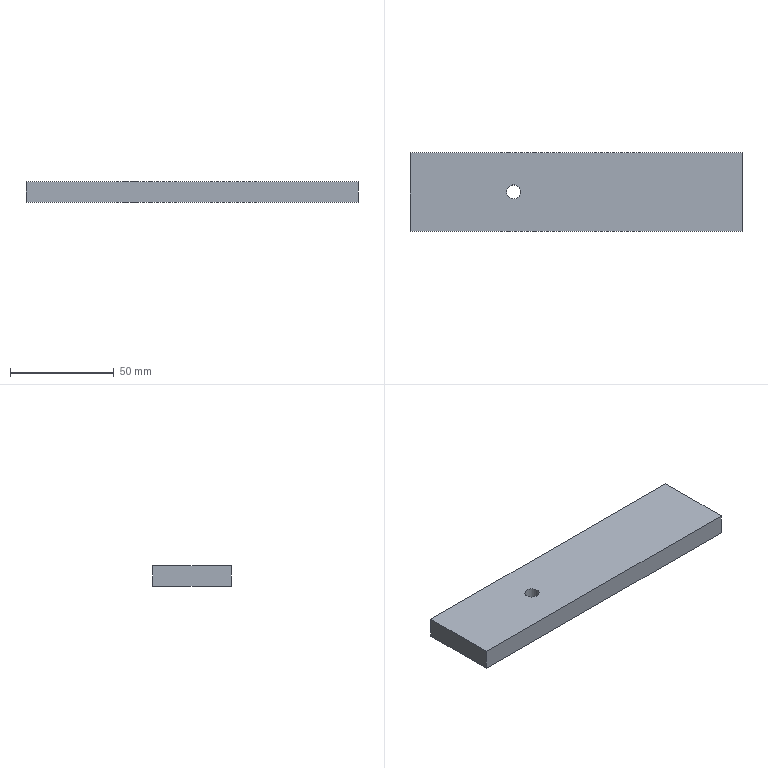Component | NX | FIXED_PLATE_11 | 1 solid | 7 faces | box 160 x 38 x 10 mm | volume 60437 mm3 | plane 6 | cylinder 1 | commonest cylinder face diameters 6.8 x1
STEP:
#1=CARTESIAN_POINT('',(0.,0.,0.));
#2=DIRECTION('',(0.,0.,1.));
#3=DIRECTION('',(1.,0.,0.));
#4=AXIS2_PLACEMENT_3D('',#1,#2,#3);
#5=CARTESIAN_POINT('',(1356.736,1345.,801.574));
#6=VERTEX_POINT('',#5);
#7=CARTESIAN_POINT('',(1356.736,1307.,801.574));
#8=VERTEX_POINT('',#7);
#9=CARTESIAN_POINT('',(1356.736,1345.,801.574));
#10=DIRECTION('',(0.,-1.,0.));
#11=VECTOR('',#10,1.);
#12=LINE('',#9,#11);
#13=CARTESIAN_POINT('',(1356.736,1345.,791.574));
#14=DIRECTION('',(-1.,0.,0.));
#15=DIRECTION('',(0.,0.,1.));
#16=AXIS2_PLACEMENT_3D('',#13,#14,#15);
#17=PLANE('',#16);
#18=CARTESIAN_POINT('',(10.,0.));
#19=DIRECTION('',(0.,-1.));
#20=VECTOR('',#19,1.);
#21=LINE('',#18,#20);
#22=(GEOMETRIC_REPRESENTATION_CONTEXT(2)PARAMETRIC_REPRESENTATION_CONTEXT()REPRESENTATION_CONTEXT('',''));
#23=DEFINITIONAL_REPRESENTATION('',(#21),#22);
#24=PCURVE('',#17,#23);
#25=CARTESIAN_POINT('',(1406.736,1326.,801.574));
#26=DIRECTION('',(0.,0.,1.));
#27=DIRECTION('',(1.,0.,0.));
#28=AXIS2_PLACEMENT_3D('',#25,#26,#27);
#29=PLANE('',#28);
#30=CARTESIAN_POINT('',(-50.,19.));
#31=DIRECTION('',(0.,-1.));
#32=VECTOR('',#31,1.);
#33=LINE('',#30,#32);
#34=(GEOMETRIC_REPRESENTATION_CONTEXT(2)PARAMETRIC_REPRESENTATION_CONTEXT()REPRESENTATION_CONTEXT('',''));
#35=DEFINITIONAL_REPRESENTATION('',(#33),#34);
#36=PCURVE('',#29,#35);
#37=SURFACE_CURVE('',#12,(#24,#36),.PCURVE_S1.);
#38=EDGE_CURVE('',#6,#8,#37,.T.);
#39=ORIENTED_EDGE('',*,*,#38,.F.);
#40=CARTESIAN_POINT('',(1356.736,1345.,791.574));
#41=VERTEX_POINT('',#40);
#42=CARTESIAN_POINT('',(1356.736,1345.,791.574));
#43=DIRECTION('',(0.,0.,1.));
#44=VECTOR('',#43,1.);
#45=LINE('',#42,#44);
#46=CARTESIAN_POINT('',(0.,0.));
#47=DIRECTION('',(1.,0.));
#48=VECTOR('',#47,1.);
#49=LINE('',#46,#48);
#50=(GEOMETRIC_REPRESENTATION_CONTEXT(2)PARAMETRIC_REPRESENTATION_CONTEXT()REPRESENTATION_CONTEXT('',''));
#51=DEFINITIONAL_REPRESENTATION('',(#49),#50);
#52=PCURVE('',#17,#51);
#53=CARTESIAN_POINT('',(1516.736,1345.,791.574));
#54=DIRECTION('',(0.,1.,0.));
#55=DIRECTION('',(0.,0.,1.));
#56=AXIS2_PLACEMENT_3D('',#53,#54,#55);
#57=PLANE('',#56);
#58=CARTESIAN_POINT('',(0.,-160.));
#59=DIRECTION('',(1.,0.));
#60=VECTOR('',#59,1.);
#61=LINE('',#58,#60);
#62=(GEOMETRIC_REPRESENTATION_CONTEXT(2)PARAMETRIC_REPRESENTATION_CONTEXT()REPRESENTATION_CONTEXT('',''));
#63=DEFINITIONAL_REPRESENTATION('',(#61),#62);
#64=PCURVE('',#57,#63);
#65=SURFACE_CURVE('',#45,(#52,#64),.PCURVE_S1.);
#66=EDGE_CURVE('',#41,#6,#65,.T.);
#67=ORIENTED_EDGE('',*,*,#66,.F.);
#68=CARTESIAN_POINT('',(1356.736,1307.,791.574));
#69=VERTEX_POINT('',#68);
#70=CARTESIAN_POINT('',(1356.736,1345.,791.574));
#71=DIRECTION('',(0.,-1.,0.));
#72=VECTOR('',#71,1.);
#73=LINE('',#70,#72);
#74=CARTESIAN_POINT('',(0.,0.));
#75=DIRECTION('',(0.,-1.));
#76=VECTOR('',#75,1.);
#77=LINE('',#74,#76);
#78=(GEOMETRIC_REPRESENTATION_CONTEXT(2)PARAMETRIC_REPRESENTATION_CONTEXT()REPRESENTATION_CONTEXT('',''));
#79=DEFINITIONAL_REPRESENTATION('',(#77),#78);
#80=PCURVE('',#17,#79);
#81=CARTESIAN_POINT('',(1406.736,1326.,791.574));
#82=DIRECTION('',(0.,0.,1.));
#83=DIRECTION('',(1.,0.,0.));
#84=AXIS2_PLACEMENT_3D('',#81,#82,#83);
#85=PLANE('',#84);
#86=CARTESIAN_POINT('',(-50.,19.));
#87=DIRECTION('',(0.,-1.));
#88=VECTOR('',#87,1.);
#89=LINE('',#86,#88);
#90=(GEOMETRIC_REPRESENTATION_CONTEXT(2)PARAMETRIC_REPRESENTATION_CONTEXT()REPRESENTATION_CONTEXT('',''));
#91=DEFINITIONAL_REPRESENTATION('',(#89),#90);
#92=PCURVE('',#85,#91);
#93=SURFACE_CURVE('',#73,(#80,#92),.PCURVE_S1.);
#94=EDGE_CURVE('',#41,#69,#93,.T.);
#95=ORIENTED_EDGE('',*,*,#94,.T.);
#96=CARTESIAN_POINT('',(1356.736,1307.,791.574));
#97=DIRECTION('',(0.,0.,1.));
#98=VECTOR('',#97,1.);
#99=LINE('',#96,#98);
#100=CARTESIAN_POINT('',(0.,-38.));
#101=DIRECTION('',(1.,0.));
#102=VECTOR('',#101,1.);
#103=LINE('',#100,#102);
#104=(GEOMETRIC_REPRESENTATION_CONTEXT(2)PARAMETRIC_REPRESENTATION_CONTEXT()REPRESENTATION_CONTEXT('',''));
#105=DEFINITIONAL_REPRESENTATION('',(#103),#104);
#106=PCURVE('',#17,#105);
#107=CARTESIAN_POINT('',(1356.736,1307.,791.574));
#108=DIRECTION('',(-0.,-1.,0.));
#109=DIRECTION('',(1.,-0.,0.));
#110=AXIS2_PLACEMENT_3D('',#107,#108,#109);
#111=PLANE('',#110);
#112=CARTESIAN_POINT('',(0.,0.));
#113=DIRECTION('',(0.,1.));
#114=VECTOR('',#113,1.);
#115=LINE('',#112,#114);
#116=(GEOMETRIC_REPRESENTATION_CONTEXT(2)PARAMETRIC_REPRESENTATION_CONTEXT()REPRESENTATION_CONTEXT('',''));
#117=DEFINITIONAL_REPRESENTATION('',(#115),#116);
#118=PCURVE('',#111,#117);
#119=SURFACE_CURVE('',#99,(#106,#118),.PCURVE_S1.);
#120=EDGE_CURVE('',#69,#8,#119,.T.);
#121=ORIENTED_EDGE('',*,*,#120,.T.);
#122=EDGE_LOOP('',(#39,#67,#95,#121));
#123=FACE_BOUND('',#122,.T.);
#124=ADVANCED_FACE('',(#123),#17,.T.);
#125=CARTESIAN_POINT('',(1516.736,1307.,801.574));
#126=VERTEX_POINT('',#125);
#127=CARTESIAN_POINT('',(1356.736,1307.,801.574));
#128=DIRECTION('',(1.,-0.,0.));
#129=VECTOR('',#128,1.);
#130=LINE('',#127,#129);
#131=CARTESIAN_POINT('',(0.,10.));
#132=DIRECTION('',(1.,0.));
#133=VECTOR('',#132,1.);
#134=LINE('',#131,#133);
#135=(GEOMETRIC_REPRESENTATION_CONTEXT(2)PARAMETRIC_REPRESENTATION_CONTEXT()REPRESENTATION_CONTEXT('',''));
#136=DEFINITIONAL_REPRESENTATION('',(#134),#135);
#137=PCURVE('',#111,#136);
#138=CARTESIAN_POINT('',(-50.,-19.));
#139=DIRECTION('',(1.,-0.));
#140=VECTOR('',#139,1.);
#141=LINE('',#138,#140);
#142=(GEOMETRIC_REPRESENTATION_CONTEXT(2)PARAMETRIC_REPRESENTATION_CONTEXT()REPRESENTATION_CONTEXT('',''));
#143=DEFINITIONAL_REPRESENTATION('',(#141),#142);
#144=PCURVE('',#29,#143);
#145=SURFACE_CURVE('',#130,(#137,#144),.PCURVE_S1.);
#146=EDGE_CURVE('',#8,#126,#145,.T.);
#147=ORIENTED_EDGE('',*,*,#146,.F.);
#148=ORIENTED_EDGE('',*,*,#120,.F.);
#149=CARTESIAN_POINT('',(1516.736,1307.,791.574));
#150=VERTEX_POINT('',#149);
#151=CARTESIAN_POINT('',(1356.736,1307.,791.574));
#152=DIRECTION('',(1.,-0.,0.));
#153=VECTOR('',#152,1.);
#154=LINE('',#151,#153);
#155=CARTESIAN_POINT('',(0.,0.));
#156=DIRECTION('',(1.,0.));
#157=VECTOR('',#156,1.);
#158=LINE('',#155,#157);
#159=(GEOMETRIC_REPRESENTATION_CONTEXT(2)PARAMETRIC_REPRESENTATION_CONTEXT()REPRESENTATION_CONTEXT('',''));
#160=DEFINITIONAL_REPRESENTATION('',(#158),#159);
#161=PCURVE('',#111,#160);
#162=CARTESIAN_POINT('',(-50.,-19.));
#163=DIRECTION('',(1.,-0.));
#164=VECTOR('',#163,1.);
#165=LINE('',#162,#164);
#166=(GEOMETRIC_REPRESENTATION_CONTEXT(2)PARAMETRIC_REPRESENTATION_CONTEXT()REPRESENTATION_CONTEXT('',''));
#167=DEFINITIONAL_REPRESENTATION('',(#165),#166);
#168=PCURVE('',#85,#167);
#169=SURFACE_CURVE('',#154,(#161,#168),.PCURVE_S1.);
#170=EDGE_CURVE('',#69,#150,#169,.T.);
#171=ORIENTED_EDGE('',*,*,#170,.T.);
#172=CARTESIAN_POINT('',(1516.736,1307.,791.574));
#173=DIRECTION('',(0.,0.,1.));
#174=VECTOR('',#173,1.);
#175=LINE('',#172,#174);
#176=CARTESIAN_POINT('',(160.,0.));
#177=DIRECTION('',(0.,1.));
#178=VECTOR('',#177,1.);
#179=LINE('',#176,#178);
#180=(GEOMETRIC_REPRESENTATION_CONTEXT(2)PARAMETRIC_REPRESENTATION_CONTEXT()REPRESENTATION_CONTEXT('',''));
#181=DEFINITIONAL_REPRESENTATION('',(#179),#180);
#182=PCURVE('',#111,#181);
#183=CARTESIAN_POINT('',(1516.736,1307.,791.574));
#184=DIRECTION('',(1.,0.,0.));
#185=DIRECTION('',(0.,0.,-1.));
#186=AXIS2_PLACEMENT_3D('',#183,#184,#185);
#187=PLANE('',#186);
#188=CARTESIAN_POINT('',(0.,0.));
#189=DIRECTION('',(-1.,0.));
#190=VECTOR('',#189,1.);
#191=LINE('',#188,#190);
#192=(GEOMETRIC_REPRESENTATION_CONTEXT(2)PARAMETRIC_REPRESENTATION_CONTEXT()REPRESENTATION_CONTEXT('',''));
#193=DEFINITIONAL_REPRESENTATION('',(#191),#192);
#194=PCURVE('',#187,#193);
#195=SURFACE_CURVE('',#175,(#182,#194),.PCURVE_S1.);
#196=EDGE_CURVE('',#150,#126,#195,.T.);
#197=ORIENTED_EDGE('',*,*,#196,.T.);
#198=EDGE_LOOP('',(#147,#148,#171,#197));
#199=FACE_BOUND('',#198,.T.);
#200=ADVANCED_FACE('',(#199),#111,.T.);
#201=CARTESIAN_POINT('',(1516.736,1345.,801.574));
#202=VERTEX_POINT('',#201);
#203=CARTESIAN_POINT('',(1516.736,1307.,801.574));
#204=DIRECTION('',(0.,1.,0.));
#205=VECTOR('',#204,1.);
#206=LINE('',#203,#205);
#207=CARTESIAN_POINT('',(-10.,0.));
#208=DIRECTION('',(0.,1.));
#209=VECTOR('',#208,1.);
#210=LINE('',#207,#209);
#211=(GEOMETRIC_REPRESENTATION_CONTEXT(2)PARAMETRIC_REPRESENTATION_CONTEXT()REPRESENTATION_CONTEXT('',''));
#212=DEFINITIONAL_REPRESENTATION('',(#210),#211);
#213=PCURVE('',#187,#212);
#214=CARTESIAN_POINT('',(110.,-19.));
#215=DIRECTION('',(0.,1.));
#216=VECTOR('',#215,1.);
#217=LINE('',#214,#216);
#218=(GEOMETRIC_REPRESENTATION_CONTEXT(2)PARAMETRIC_REPRESENTATION_CONTEXT()REPRESENTATION_CONTEXT('',''));
#219=DEFINITIONAL_REPRESENTATION('',(#217),#218);
#220=PCURVE('',#29,#219);
#221=SURFACE_CURVE('',#206,(#213,#220),.PCURVE_S1.);
#222=EDGE_CURVE('',#126,#202,#221,.T.);
#223=ORIENTED_EDGE('',*,*,#222,.F.);
#224=ORIENTED_EDGE('',*,*,#196,.F.);
#225=CARTESIAN_POINT('',(1516.736,1345.,791.574));
#226=VERTEX_POINT('',#225);
#227=CARTESIAN_POINT('',(1516.736,1307.,791.574));
#228=DIRECTION('',(0.,1.,0.));
#229=VECTOR('',#228,1.);
#230=LINE('',#227,#229);
#231=CARTESIAN_POINT('',(0.,0.));
#232=DIRECTION('',(0.,1.));
#233=VECTOR('',#232,1.);
#234=LINE('',#231,#233);
#235=(GEOMETRIC_REPRESENTATION_CONTEXT(2)PARAMETRIC_REPRESENTATION_CONTEXT()REPRESENTATION_CONTEXT('',''));
#236=DEFINITIONAL_REPRESENTATION('',(#234),#235);
#237=PCURVE('',#187,#236);
#238=CARTESIAN_POINT('',(110.,-19.));
#239=DIRECTION('',(0.,1.));
#240=VECTOR('',#239,1.);
#241=LINE('',#238,#240);
#242=(GEOMETRIC_REPRESENTATION_CONTEXT(2)PARAMETRIC_REPRESENTATION_CONTEXT()REPRESENTATION_CONTEXT('',''));
#243=DEFINITIONAL_REPRESENTATION('',(#241),#242);
#244=PCURVE('',#85,#243);
#245=SURFACE_CURVE('',#230,(#237,#244),.PCURVE_S1.);
#246=EDGE_CURVE('',#150,#226,#245,.T.);
#247=ORIENTED_EDGE('',*,*,#246,.T.);
#248=CARTESIAN_POINT('',(1516.736,1345.,791.574));
#249=DIRECTION('',(0.,0.,1.));
#250=VECTOR('',#249,1.);
#251=LINE('',#248,#250);
#252=CARTESIAN_POINT('',(0.,38.));
#253=DIRECTION('',(-1.,0.));
#254=VECTOR('',#253,1.);
#255=LINE('',#252,#254);
#256=(GEOMETRIC_REPRESENTATION_CONTEXT(2)PARAMETRIC_REPRESENTATION_CONTEXT()REPRESENTATION_CONTEXT('',''));
#257=DEFINITIONAL_REPRESENTATION('',(#255),#256);
#258=PCURVE('',#187,#257);
#259=CARTESIAN_POINT('',(0.,0.));
#260=DIRECTION('',(1.,0.));
#261=VECTOR('',#260,1.);
#262=LINE('',#259,#261);
#263=(GEOMETRIC_REPRESENTATION_CONTEXT(2)PARAMETRIC_REPRESENTATION_CONTEXT()REPRESENTATION_CONTEXT('',''));
#264=DEFINITIONAL_REPRESENTATION('',(#262),#263);
#265=PCURVE('',#57,#264);
#266=SURFACE_CURVE('',#251,(#258,#265),.PCURVE_S1.);
#267=EDGE_CURVE('',#226,#202,#266,.T.);
#268=ORIENTED_EDGE('',*,*,#267,.T.);
#269=EDGE_LOOP('',(#223,#224,#247,#268));
#270=FACE_BOUND('',#269,.T.);
#271=ADVANCED_FACE('',(#270),#187,.T.);
#272=CARTESIAN_POINT('',(1516.736,1345.,801.574));
#273=DIRECTION('',(-1.,0.,0.));
#274=VECTOR('',#273,1.);
#275=LINE('',#272,#274);
#276=CARTESIAN_POINT('',(10.,0.));
#277=DIRECTION('',(0.,-1.));
#278=VECTOR('',#277,1.);
#279=LINE('',#276,#278);
#280=(GEOMETRIC_REPRESENTATION_CONTEXT(2)PARAMETRIC_REPRESENTATION_CONTEXT()REPRESENTATION_CONTEXT('',''));
#281=DEFINITIONAL_REPRESENTATION('',(#279),#280);
#282=PCURVE('',#57,#281);
#283=CARTESIAN_POINT('',(110.,19.));
#284=DIRECTION('',(-1.,0.));
#285=VECTOR('',#284,1.);
#286=LINE('',#283,#285);
#287=(GEOMETRIC_REPRESENTATION_CONTEXT(2)PARAMETRIC_REPRESENTATION_CONTEXT()REPRESENTATION_CONTEXT('',''));
#288=DEFINITIONAL_REPRESENTATION('',(#286),#287);
#289=PCURVE('',#29,#288);
#290=SURFACE_CURVE('',#275,(#282,#289),.PCURVE_S1.);
#291=EDGE_CURVE('',#202,#6,#290,.T.);
#292=ORIENTED_EDGE('',*,*,#291,.F.);
#293=ORIENTED_EDGE('',*,*,#267,.F.);
#294=CARTESIAN_POINT('',(1516.736,1345.,791.574));
#295=DIRECTION('',(-1.,0.,0.));
#296=VECTOR('',#295,1.);
#297=LINE('',#294,#296);
#298=CARTESIAN_POINT('',(0.,0.));
#299=DIRECTION('',(0.,-1.));
#300=VECTOR('',#299,1.);
#301=LINE('',#298,#300);
#302=(GEOMETRIC_REPRESENTATION_CONTEXT(2)PARAMETRIC_REPRESENTATION_CONTEXT()REPRESENTATION_CONTEXT('',''));
#303=DEFINITIONAL_REPRESENTATION('',(#301),#302);
#304=PCURVE('',#57,#303);
#305=CARTESIAN_POINT('',(110.,19.));
#306=DIRECTION('',(-1.,0.));
#307=VECTOR('',#306,1.);
#308=LINE('',#305,#307);
#309=(GEOMETRIC_REPRESENTATION_CONTEXT(2)PARAMETRIC_REPRESENTATION_CONTEXT()REPRESENTATION_CONTEXT('',''));
#310=DEFINITIONAL_REPRESENTATION('',(#308),#309);
#311=PCURVE('',#85,#310);
#312=SURFACE_CURVE('',#297,(#304,#311),.PCURVE_S1.);
#313=EDGE_CURVE('',#226,#41,#312,.T.);
#314=ORIENTED_EDGE('',*,*,#313,.T.);
#315=ORIENTED_EDGE('',*,*,#66,.T.);
#316=EDGE_LOOP('',(#292,#293,#314,#315));
#317=FACE_BOUND('',#316,.T.);
#318=ADVANCED_FACE('',(#317),#57,.T.);
#319=CARTESIAN_POINT('',(1410.136,1326.,791.574));
#320=VERTEX_POINT('',#319);
#321=CARTESIAN_POINT('',(1406.736,1326.,791.574));
#322=DIRECTION('',(0.,0.,1.));
#323=DIRECTION('',(1.,0.,0.));
#324=AXIS2_PLACEMENT_3D('',#321,#322,#323);
#325=CIRCLE('',#324,3.4);
#326=CARTESIAN_POINT('',(1406.736,1326.,791.574));
#327=DIRECTION('',(0.,0.,1.));
#328=DIRECTION('',(1.,0.,0.));
#329=AXIS2_PLACEMENT_3D('',#326,#327,#328);
#330=CYLINDRICAL_SURFACE('',#329,3.4);
#331=CARTESIAN_POINT('',(0.,0.));
#332=DIRECTION('',(1.,0.));
#333=VECTOR('',#332,1.);
#334=LINE('',#331,#333);
#335=(GEOMETRIC_REPRESENTATION_CONTEXT(2)PARAMETRIC_REPRESENTATION_CONTEXT()REPRESENTATION_CONTEXT('',''));
#336=DEFINITIONAL_REPRESENTATION('',(#334),#335);
#337=PCURVE('',#330,#336);
#338=CARTESIAN_POINT('',(0.,0.));
#339=DIRECTION('',(1.,0.));
#340=AXIS2_PLACEMENT_2D('',#338,#339);
#341=CIRCLE('',#340,3.4);
#342=(GEOMETRIC_REPRESENTATION_CONTEXT(2)PARAMETRIC_REPRESENTATION_CONTEXT()REPRESENTATION_CONTEXT('',''));
#343=DEFINITIONAL_REPRESENTATION('',(#341),#342);
#344=PCURVE('',#85,#343);
#345=SURFACE_CURVE('',#325,(#337,#344),.PCURVE_S1.);
#346=EDGE_CURVE('',#320,#320,#345,.T.);
#347=ORIENTED_EDGE('',*,*,#346,.T.);
#348=CARTESIAN_POINT('',(1410.136,1326.,801.574));
#349=VERTEX_POINT('',#348);
#350=CARTESIAN_POINT('',(1410.136,1326.,791.574));
#351=CARTESIAN_POINT('',(1410.136,1326.,801.574));
#352=B_SPLINE_CURVE_WITH_KNOTS('',1,(#350,#351),.UNSPECIFIED.,.F.,.F.,(2,2),(0.,10.),.PIECEWISE_BEZIER_KNOTS.);
#353=CARTESIAN_POINT('',(6.283,0.));
#354=DIRECTION('',(0.,1.));
#355=VECTOR('',#354,1.);
#356=LINE('',#353,#355);
#357=(GEOMETRIC_REPRESENTATION_CONTEXT(2)PARAMETRIC_REPRESENTATION_CONTEXT()REPRESENTATION_CONTEXT('',''));
#358=DEFINITIONAL_REPRESENTATION('',(#356),#357);
#359=PCURVE('',#330,#358);
#360=CARTESIAN_POINT('',(0.,0.));
#361=DIRECTION('',(0.,1.));
#362=VECTOR('',#361,1.);
#363=LINE('',#360,#362);
#364=(GEOMETRIC_REPRESENTATION_CONTEXT(2)PARAMETRIC_REPRESENTATION_CONTEXT()REPRESENTATION_CONTEXT('',''));
#365=DEFINITIONAL_REPRESENTATION('',(#363),#364);
#366=PCURVE('',#330,#365);
#367=SEAM_CURVE('',#352,(#359,#366),.PCURVE_S1.);
#368=EDGE_CURVE('',#320,#349,#367,.T.);
#369=ORIENTED_EDGE('',*,*,#368,.T.);
#370=CARTESIAN_POINT('',(1406.736,1326.,801.574));
#371=DIRECTION('',(0.,0.,1.));
#372=DIRECTION('',(1.,0.,0.));
#373=AXIS2_PLACEMENT_3D('',#370,#371,#372);
#374=CIRCLE('',#373,3.4);
#375=CARTESIAN_POINT('',(0.,10.));
#376=DIRECTION('',(1.,0.));
#377=VECTOR('',#376,1.);
#378=LINE('',#375,#377);
#379=(GEOMETRIC_REPRESENTATION_CONTEXT(2)PARAMETRIC_REPRESENTATION_CONTEXT()REPRESENTATION_CONTEXT('',''));
#380=DEFINITIONAL_REPRESENTATION('',(#378),#379);
#381=PCURVE('',#330,#380);
#382=CARTESIAN_POINT('',(0.,0.));
#383=DIRECTION('',(1.,0.));
#384=AXIS2_PLACEMENT_2D('',#382,#383);
#385=CIRCLE('',#384,3.4);
#386=(GEOMETRIC_REPRESENTATION_CONTEXT(2)PARAMETRIC_REPRESENTATION_CONTEXT()REPRESENTATION_CONTEXT('',''));
#387=DEFINITIONAL_REPRESENTATION('',(#385),#386);
#388=PCURVE('',#29,#387);
#389=SURFACE_CURVE('',#374,(#381,#388),.PCURVE_S1.);
#390=EDGE_CURVE('',#349,#349,#389,.T.);
#391=ORIENTED_EDGE('',*,*,#390,.F.);
#392=ORIENTED_EDGE('',*,*,#368,.F.);
#393=EDGE_LOOP('',(#347,#369,#391,#392));
#394=FACE_BOUND('',#393,.F.);
#395=ADVANCED_FACE('',(#394),#330,.F.);
#396=ORIENTED_EDGE('',*,*,#94,.F.);
#397=ORIENTED_EDGE('',*,*,#313,.F.);
#398=ORIENTED_EDGE('',*,*,#246,.F.);
#399=ORIENTED_EDGE('',*,*,#170,.F.);
#400=EDGE_LOOP('',(#396,#397,#398,#399));
#401=FACE_BOUND('',#400,.T.);
#402=ORIENTED_EDGE('',*,*,#346,.T.);
#403=EDGE_LOOP('',(#402));
#404=FACE_BOUND('',#403,.T.);
#405=ADVANCED_FACE('',(#401,#404),#85,.F.);
#406=ORIENTED_EDGE('',*,*,#38,.T.);
#407=ORIENTED_EDGE('',*,*,#146,.T.);
#408=ORIENTED_EDGE('',*,*,#222,.T.);
#409=ORIENTED_EDGE('',*,*,#291,.T.);
#410=EDGE_LOOP('',(#406,#407,#408,#409));
#411=FACE_BOUND('',#410,.T.);
#412=ORIENTED_EDGE('',*,*,#390,.F.);
#413=EDGE_LOOP('',(#412));
#414=FACE_BOUND('',#413,.T.);
#415=ADVANCED_FACE('',(#411,#414),#29,.T.);
#416=CLOSED_SHELL('',(#124,#200,#271,#318,#395,#405,#415));
#417=MANIFOLD_SOLID_BREP('',#416);
#418=(LENGTH_UNIT()NAMED_UNIT(*)SI_UNIT(.MILLI.,.METRE.));
#419=UNCERTAINTY_MEASURE_WITH_UNIT(LENGTH_MEASURE(0.000002),#418,'','');
#420=(NAMED_UNIT(*)PLANE_ANGLE_UNIT()SI_UNIT($,.RADIAN.));
#421=(NAMED_UNIT(*)SI_UNIT($,.STERADIAN.)SOLID_ANGLE_UNIT());
#422=(GEOMETRIC_REPRESENTATION_CONTEXT(3)GLOBAL_UNCERTAINTY_ASSIGNED_CONTEXT((#419))GLOBAL_UNIT_ASSIGNED_CONTEXT((#418,#420,#421))REPRESENTATION_CONTEXT('',''));
#423=ADVANCED_BREP_SHAPE_REPRESENTATION('',(#4,#417),#422);